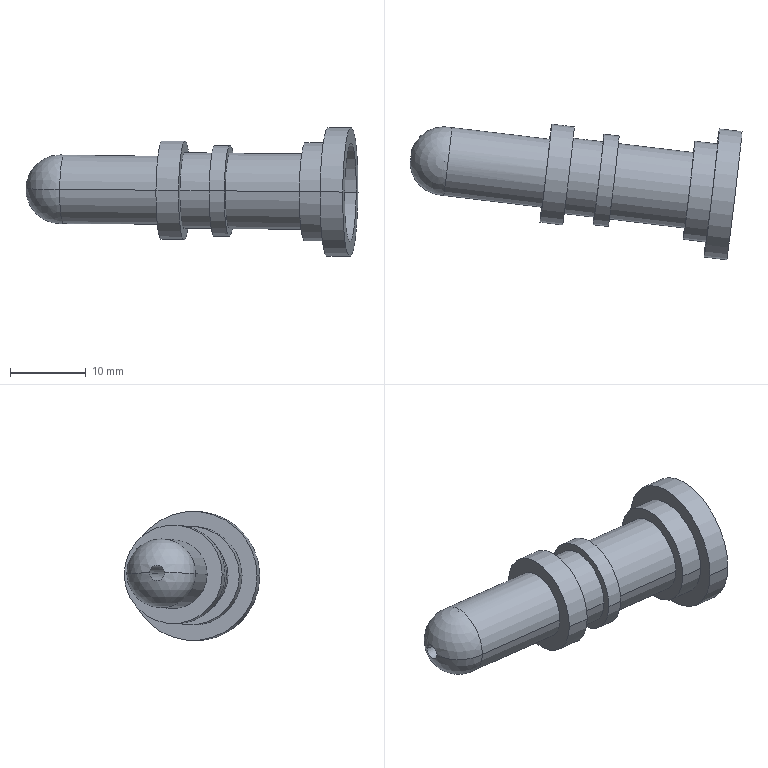Component | SolidWorks | Part12-1 | 1 solid | 29 faces | box 43.71 x 17.85 x 17.03 mm | volume 3533 mm3 | cylinder 18 | plane 9 | sphere 2 | commonest cylinder face diameters 13 x6 10 x4 2 x2 9 x2 12 x2 17 x2 | material 45
build123d program:
from build123d import *

# Parameters (mm, degrees)
SKETCH1_R                = 5
BOSS_EXTRUDE1_DEPTH      = 3
SKETCH2_R                = 6.5
BOSS_EXTRUDE2_DEPTH      = 4
BOSS_EXTRUDE3_DEPTH      = 2
BOSS_EXTRUDE3_DEPTH_BACK = 1
SKETCH3_R                = 8.5
SKETCH3_R_2              = 6.5
SKETCH4_R                = 5
BOSS_EXTRUDE4_DEPTH      = 9
SKETCH5_R                = 6
BOSS_EXTRUDE5_DEPTH      = 2
SKETCH7_R                = 5
BOSS_EXTRUDE6_DEPTH      = 4
BOSS_EXTRUDE7_START      = 3
SKETCH8_R                = 6.5
BOSS_EXTRUDE7_DEPTH      = 3
SKETCH10_R               = 4.5
BOSS_EXTRUDE8_DEPTH      = 13
DOME1_FACE_RADIUS        = 4.5
DOME1_HEIGHT             = 5
SKETCH11_R               = 1
CUT_EXTRUDE1_DEPTH       = 26


with BuildPart() as part:
    # Sketch1 → Boss-Extrude1 (new body)
    with BuildSketch(Plane.XY):
        with Locations((3, 0)):
            Circle(SKETCH1_R)
    extrude(amount=-BOSS_EXTRUDE1_DEPTH)

    # Sketch2 → Boss-Extrude2 (add)
    with BuildSketch(Plane.XY):
        with Locations((3, 0)):
            Circle(SKETCH2_R)
    extrude(amount=BOSS_EXTRUDE2_DEPTH)

    # Sketch3 → Boss-Extrude3 (add, two sides: drawn at the far end of the back side and taken through both)
    with BuildSketch(Plane.XY.offset(4).offset(-BOSS_EXTRUDE3_DEPTH_BACK)):
        with Locations((3, 0)):
            Circle(SKETCH3_R)
        with Locations((3, 0)):
            Circle(SKETCH3_R_2, mode=Mode.SUBTRACT)
    extrude(amount=BOSS_EXTRUDE3_DEPTH + BOSS_EXTRUDE3_DEPTH_BACK)

    # Sketch4 → Boss-Extrude4 (add)
    with BuildSketch(Plane(origin=(0, 0, -3), x_dir=(-1, 0, 0), z_dir=(0, 0, -1))):
        with Locations(Location((-3, 0, 0), (0, 0, 180))):
            Circle(SKETCH4_R)
    extrude(amount=BOSS_EXTRUDE4_DEPTH)

    # Sketch5 → Boss-Extrude5 (add)
    with BuildSketch(Plane(origin=(0, 0, -12), x_dir=(-1, 0, 0), z_dir=(0, 0, -1))):
        with Locations((-3, 0)):
            Circle(SKETCH5_R)
    extrude(amount=-BOSS_EXTRUDE5_DEPTH)

    # Sketch7 → Boss-Extrude6 (add)
    with BuildSketch(Plane(origin=(0, 0, -12), x_dir=(-1, 0, 0), z_dir=(0, 0, -1))):
        with Locations(Location((-3, 0, 0), (0, 0, 180))):
            Circle(SKETCH7_R)
    extrude(amount=BOSS_EXTRUDE6_DEPTH)

    # Sketch8 → Boss-Extrude7 (add)
    with BuildSketch(Plane(origin=(0, 0, -16), x_dir=(-1, 0, 0), z_dir=(0, 0, -1)).offset(BOSS_EXTRUDE7_START)):
        with Locations(Location((-3, 0, 0), (0, 0, 180))):
            Circle(SKETCH8_R)
    extrude(amount=-BOSS_EXTRUDE7_DEPTH)

    # Sketch10 → Boss-Extrude8 (add)
    with BuildSketch(Plane(origin=(0, 0, -19), x_dir=(-1, 0, 0), z_dir=(0, 0, -1))):
        with Locations((-3, 0)):
            Circle(SKETCH10_R)
    extrude(amount=BOSS_EXTRUDE8_DEPTH)

    # Dome1: a dome of height H over a round flat face of radius A is a cap of a sphere of radius (A * A + H * H) / (2 * H)
    dome1_r = (DOME1_FACE_RADIUS * DOME1_FACE_RADIUS + DOME1_HEIGHT * DOME1_HEIGHT) / (2 * DOME1_HEIGHT)
    dome1_base = Plane((3, 0, -32), z_dir=(0, 0, -1))
    with Locations(dome1_base.offset(DOME1_HEIGHT - dome1_r)):
        dome1_ball = Sphere(dome1_r, mode=Mode.PRIVATE)
    add(split(dome1_ball, bisect_by=dome1_base, keep=Keep.TOP, mode=Mode.PRIVATE))

    # Sketch11 → Cut-Extrude1 (cut)
    with BuildSketch(Plane(origin=(0, 0, -19), x_dir=(-1, 0, 0), z_dir=(0, 0, -1))):
        with Locations(Location((-3, 0, 0), (0, 0, 180))):
            Circle(SKETCH11_R)
    extrude(amount=CUT_EXTRUDE1_DEPTH, mode=Mode.SUBTRACT)


solid = part.part

# Placed as in the assembly
solid = solid.moved(Location((7.17, 63.338, -1.925), (94.698, 83.182, -4.568)))
STEP:
#1=COLOUR_RGB('',0.7922,0.8196,0.9333);
#2=FILL_AREA_STYLE_COLOUR('',#1);
#3=FILL_AREA_STYLE('',(#2));
#4=SURFACE_STYLE_FILL_AREA(#3);
#5=SURFACE_SIDE_STYLE('',(#4));
#6=SURFACE_STYLE_USAGE(.BOTH.,#5);
#7=PRESENTATION_STYLE_ASSIGNMENT((#6));
#8=CARTESIAN_POINT('',(-1.141,2.822,-0.0615));
#9=VERTEX_POINT('',#8);
#10=CARTESIAN_POINT('',(-1.15,2.744,-0.06141));
#11=VERTEX_POINT('',#10);
#12=CARTESIAN_POINT('',(-1.146,2.783,-0.06145));
#13=DIRECTION('',(0.9929,-0.1183,-0.009724));
#14=DIRECTION('',(-0.1183,-0.993,0.001159));
#15=AXIS2_PLACEMENT_3D('',#12,#13,#14);
#16=CIRCLE('',#15,0.03937);
#17=EDGE_CURVE('',#9,#11,#16,.T.);
#18=ORIENTED_EDGE('',*,*,#17,.F.);
#19=CARTESIAN_POINT('',(-0.4418,2.738,-0.06835));
#20=VERTEX_POINT('',#19);
#21=CARTESIAN_POINT('',(-1.458,2.86,-0.05839));
#22=DIRECTION('',(0.9929,-0.1183,-0.009724));
#23=VECTOR('',#22,39.37);
#24=LINE('',#21,#23);
#25=EDGE_CURVE('',#9,#20,#24,.T.);
#26=ORIENTED_EDGE('',*,*,#25,.T.);
#27=CARTESIAN_POINT('',(-0.4511,2.66,-0.06826));
#28=VERTEX_POINT('',#27);
#29=CARTESIAN_POINT('',(-0.4465,2.699,-0.0683));
#30=DIRECTION('',(-0.9929,0.1183,0.009724));
#31=DIRECTION('',(0.1183,0.993,-0.001159));
#32=AXIS2_PLACEMENT_3D('',#29,#30,#31);
#33=CIRCLE('',#32,0.03937);
#34=EDGE_CURVE('',#28,#20,#33,.T.);
#35=ORIENTED_EDGE('',*,*,#34,.F.);
#36=CARTESIAN_POINT('',(-1.468,2.781,-0.0583));
#37=DIRECTION('',(0.9929,-0.1183,-0.009724));
#38=VECTOR('',#37,39.37);
#39=LINE('',#36,#38);
#40=EDGE_CURVE('',#11,#28,#39,.T.);
#41=ORIENTED_EDGE('',*,*,#40,.F.);
#42=EDGE_LOOP('',(#18,#26,#35,#41));
#43=FACE_OUTER_BOUND('',#42,.T.);
#44=CARTESIAN_POINT('',(-1.463,2.821,-0.05835));
#45=DIRECTION('',(0.9929,-0.1183,-0.009724));
#46=DIRECTION('',(-0.1183,-0.993,0.001159));
#47=AXIS2_PLACEMENT_3D('',#44,#45,#46);
#48=CYLINDRICAL_SURFACE('',#47,0.03937);
#49=ADVANCED_FACE('',(#43),#48,.F.);
#50=CARTESIAN_POINT('',(-0.9337,2.936,-0.06353));
#51=VERTEX_POINT('',#50);
#52=CARTESIAN_POINT('',(-0.9756,2.584,-0.06312));
#53=VERTEX_POINT('',#52);
#54=CARTESIAN_POINT('',(-0.9547,2.76,-0.06333));
#55=DIRECTION('',(-0.9929,0.1183,0.009724));
#56=DIRECTION('',(0.1183,0.993,-0.001159));
#57=AXIS2_PLACEMENT_3D('',#54,#55,#56);
#58=CIRCLE('',#57,0.1772);
#59=EDGE_CURVE('',#51,#53,#58,.T.);
#60=ORIENTED_EDGE('',*,*,#59,.F.);
#61=CARTESIAN_POINT('',(-0.4255,2.875,-0.06851));
#62=VERTEX_POINT('',#61);
#63=CARTESIAN_POINT('',(-0.9337,2.936,-0.06353));
#64=DIRECTION('',(0.9929,-0.1183,-0.009724));
#65=VECTOR('',#64,39.37);
#66=LINE('',#63,#65);
#67=EDGE_CURVE('',#51,#62,#66,.T.);
#68=ORIENTED_EDGE('',*,*,#67,.T.);
#69=CARTESIAN_POINT('',(-0.4674,2.523,-0.0681));
#70=VERTEX_POINT('',#69);
#71=CARTESIAN_POINT('',(-0.4465,2.699,-0.0683));
#72=DIRECTION('',(-0.9929,0.1183,0.009724));
#73=DIRECTION('',(0.1183,0.993,-0.001159));
#74=AXIS2_PLACEMENT_3D('',#71,#72,#73);
#75=CIRCLE('',#74,0.1772);
#76=EDGE_CURVE('',#62,#70,#75,.T.);
#77=ORIENTED_EDGE('',*,*,#76,.T.);
#78=CARTESIAN_POINT('',(-0.9756,2.584,-0.06312));
#79=DIRECTION('',(0.9929,-0.1183,-0.009724));
#80=VECTOR('',#79,39.37);
#81=LINE('',#78,#80);
#82=EDGE_CURVE('',#53,#70,#81,.T.);
#83=ORIENTED_EDGE('',*,*,#82,.F.);
#84=EDGE_LOOP('',(#60,#68,#77,#83));
#85=FACE_OUTER_BOUND('',#84,.T.);
#86=CARTESIAN_POINT('',(-0.9547,2.76,-0.06333));
#87=DIRECTION('',(0.9929,-0.1183,-0.009724));
#88=DIRECTION('',(-0.1183,-0.993,0.001159));
#89=AXIS2_PLACEMENT_3D('',#86,#87,#88);
#90=CYLINDRICAL_SURFACE('',#89,0.1772);
#91=ADVANCED_FACE('',(#85),#90,.T.);
#92=CARTESIAN_POINT('',(-0.4162,2.954,-0.0686));
#93=VERTEX_POINT('',#92);
#94=CARTESIAN_POINT('',(-0.4767,2.445,-0.06801));
#95=VERTEX_POINT('',#94);
#96=CARTESIAN_POINT('',(-0.4465,2.699,-0.0683));
#97=DIRECTION('',(-0.9929,0.1183,0.009724));
#98=DIRECTION('',(0.1183,0.993,-0.001159));
#99=AXIS2_PLACEMENT_3D('',#96,#97,#98);
#100=CIRCLE('',#99,0.2559);
#101=EDGE_CURVE('',#93,#95,#100,.T.);
#102=ORIENTED_EDGE('',*,*,#101,.F.);
#103=CARTESIAN_POINT('',(-0.2989,2.94,-0.06975));
#104=VERTEX_POINT('',#103);
#105=CARTESIAN_POINT('',(-0.4162,2.954,-0.0686));
#106=DIRECTION('',(0.9929,-0.1183,-0.009724));
#107=VECTOR('',#106,39.37);
#108=LINE('',#105,#107);
#109=EDGE_CURVE('',#93,#104,#108,.T.);
#110=ORIENTED_EDGE('',*,*,#109,.T.);
#111=CARTESIAN_POINT('',(-0.3595,2.431,-0.06915));
#112=VERTEX_POINT('',#111);
#113=CARTESIAN_POINT('',(-0.3292,2.685,-0.06945));
#114=DIRECTION('',(-0.9929,0.1183,0.009724));
#115=DIRECTION('',(0.1183,0.993,-0.001159));
#116=AXIS2_PLACEMENT_3D('',#113,#114,#115);
#117=CIRCLE('',#116,0.2559);
#118=EDGE_CURVE('',#104,#112,#117,.T.);
#119=ORIENTED_EDGE('',*,*,#118,.T.);
#120=CARTESIAN_POINT('',(-0.4767,2.445,-0.06801));
#121=DIRECTION('',(0.9929,-0.1183,-0.009724));
#122=VECTOR('',#121,39.37);
#123=LINE('',#120,#122);
#124=EDGE_CURVE('',#95,#112,#123,.T.);
#125=ORIENTED_EDGE('',*,*,#124,.F.);
#126=EDGE_LOOP('',(#102,#110,#119,#125));
#127=FACE_OUTER_BOUND('',#126,.T.);
#128=CARTESIAN_POINT('',(-0.4465,2.699,-0.0683));
#129=DIRECTION('',(0.9929,-0.1183,-0.009724));
#130=DIRECTION('',(-0.1183,-0.993,0.001159));
#131=AXIS2_PLACEMENT_3D('',#128,#129,#130);
#132=CYLINDRICAL_SURFACE('',#131,0.2559);
#133=ADVANCED_FACE('',(#127),#132,.T.);
#134=CARTESIAN_POINT('',(-0.3059,2.881,-0.06968));
#135=VERTEX_POINT('',#134);
#136=CARTESIAN_POINT('',(-0.3525,2.49,-0.06922));
#137=VERTEX_POINT('',#136);
#138=CARTESIAN_POINT('',(-0.3292,2.685,-0.06945));
#139=DIRECTION('',(-0.9929,0.1183,0.009724));
#140=DIRECTION('',(0.1183,0.993,-0.001159));
#141=AXIS2_PLACEMENT_3D('',#138,#139,#140);
#142=CIRCLE('',#141,0.1969);
#143=EDGE_CURVE('',#135,#137,#142,.T.);
#144=ORIENTED_EDGE('',*,*,#143,.F.);
#145=CARTESIAN_POINT('',(-0.1495,2.862,-0.07121));
#146=VERTEX_POINT('',#145);
#147=CARTESIAN_POINT('',(-0.3059,2.881,-0.06968));
#148=DIRECTION('',(0.9929,-0.1183,-0.009724));
#149=VECTOR('',#148,39.37);
#150=LINE('',#147,#149);
#151=EDGE_CURVE('',#135,#146,#150,.T.);
#152=ORIENTED_EDGE('',*,*,#151,.T.);
#153=CARTESIAN_POINT('',(-0.1961,2.471,-0.07075));
#154=VERTEX_POINT('',#153);
#155=CARTESIAN_POINT('',(-0.1728,2.667,-0.07098));
#156=DIRECTION('',(-0.9929,0.1183,0.009724));
#157=DIRECTION('',(0.1183,0.993,-0.001159));
#158=AXIS2_PLACEMENT_3D('',#155,#156,#157);
#159=CIRCLE('',#158,0.1969);
#160=EDGE_CURVE('',#146,#154,#159,.T.);
#161=ORIENTED_EDGE('',*,*,#160,.T.);
#162=CARTESIAN_POINT('',(-0.3525,2.49,-0.06922));
#163=DIRECTION('',(0.9929,-0.1183,-0.009724));
#164=VECTOR('',#163,39.37);
#165=LINE('',#162,#164);
#166=EDGE_CURVE('',#137,#154,#165,.T.);
#167=ORIENTED_EDGE('',*,*,#166,.F.);
#168=EDGE_LOOP('',(#144,#152,#161,#167));
#169=FACE_OUTER_BOUND('',#168,.T.);
#170=CARTESIAN_POINT('',(-0.3292,2.685,-0.06945));
#171=DIRECTION('',(0.9929,-0.1183,-0.009724));
#172=DIRECTION('',(-0.1183,-0.993,0.001159));
#173=AXIS2_PLACEMENT_3D('',#170,#171,#172);
#174=CYLINDRICAL_SURFACE('',#173,0.1969);
#175=ADVANCED_FACE('',(#169),#174,.T.);
#176=CARTESIAN_POINT('',(-0.06669,2.892,-0.07202));
#177=VERTEX_POINT('',#176);
#178=CARTESIAN_POINT('',(-0.1226,2.423,-0.07147));
#179=VERTEX_POINT('',#178);
#180=CARTESIAN_POINT('',(-0.09464,2.657,-0.07175));
#181=DIRECTION('',(-0.9929,0.1183,0.009724));
#182=DIRECTION('',(0.1183,0.993,-0.001159));
#183=AXIS2_PLACEMENT_3D('',#180,#181,#182);
#184=CIRCLE('',#183,0.2362);
#185=EDGE_CURVE('',#177,#179,#184,.T.);
#186=ORIENTED_EDGE('',*,*,#185,.T.);
#187=CARTESIAN_POINT('',(-0.2008,2.432,-0.07071));
#188=VERTEX_POINT('',#187);
#189=CARTESIAN_POINT('',(-0.1226,2.423,-0.07147));
#190=DIRECTION('',(-0.9929,0.1183,0.009724));
#191=VECTOR('',#190,39.37);
#192=LINE('',#189,#191);
#193=EDGE_CURVE('',#179,#188,#192,.T.);
#194=ORIENTED_EDGE('',*,*,#193,.T.);
#195=CARTESIAN_POINT('',(-0.1449,2.901,-0.07126));
#196=VERTEX_POINT('',#195);
#197=CARTESIAN_POINT('',(-0.1728,2.667,-0.07098));
#198=DIRECTION('',(-0.9929,0.1183,0.009724));
#199=DIRECTION('',(0.1183,0.993,-0.001159));
#200=AXIS2_PLACEMENT_3D('',#197,#198,#199);
#201=CIRCLE('',#200,0.2362);
#202=EDGE_CURVE('',#196,#188,#201,.T.);
#203=ORIENTED_EDGE('',*,*,#202,.F.);
#204=CARTESIAN_POINT('',(-0.06669,2.892,-0.07202));
#205=DIRECTION('',(-0.9929,0.1183,0.009724));
#206=VECTOR('',#205,39.37);
#207=LINE('',#204,#206);
#208=EDGE_CURVE('',#177,#196,#207,.T.);
#209=ORIENTED_EDGE('',*,*,#208,.F.);
#210=EDGE_LOOP('',(#186,#194,#203,#209));
#211=FACE_OUTER_BOUND('',#210,.T.);
#212=CARTESIAN_POINT('',(-0.09464,2.657,-0.07175));
#213=DIRECTION('',(-0.9929,0.1183,0.009724));
#214=DIRECTION('',(0.1183,0.993,-0.001159));
#215=AXIS2_PLACEMENT_3D('',#212,#213,#214);
#216=CYLINDRICAL_SURFACE('',#215,0.2362);
#217=ADVANCED_FACE('',(#211),#216,.T.);
#218=CARTESIAN_POINT('',(0.4829,2.846,-0.07741));
#219=VERTEX_POINT('',#218);
#220=CARTESIAN_POINT('',(0.4224,2.338,-0.07681));
#221=VERTEX_POINT('',#220);
#222=CARTESIAN_POINT('',(0.4526,2.592,-0.07711));
#223=DIRECTION('',(0.9929,-0.1183,-0.009724));
#224=DIRECTION('',(-0.1183,-0.993,0.001159));
#225=AXIS2_PLACEMENT_3D('',#222,#223,#224);
#226=CIRCLE('',#225,0.2559);
#227=EDGE_CURVE('',#219,#221,#226,.T.);
#228=ORIENTED_EDGE('',*,*,#227,.F.);
#229=CARTESIAN_POINT('',(0.5611,2.837,-0.07817));
#230=VERTEX_POINT('',#229);
#231=CARTESIAN_POINT('',(0.4438,2.851,-0.07702));
#232=DIRECTION('',(0.9929,-0.1183,-0.009724));
#233=VECTOR('',#232,39.37);
#234=LINE('',#231,#233);
#235=EDGE_CURVE('',#219,#230,#234,.T.);
#236=ORIENTED_EDGE('',*,*,#235,.T.);
#237=CARTESIAN_POINT('',(0.5005,2.329,-0.07758));
#238=VERTEX_POINT('',#237);
#239=CARTESIAN_POINT('',(0.5308,2.583,-0.07787));
#240=DIRECTION('',(0.9929,-0.1183,-0.009724));
#241=DIRECTION('',(-0.1183,-0.993,0.001159));
#242=AXIS2_PLACEMENT_3D('',#239,#240,#241);
#243=CIRCLE('',#242,0.2559);
#244=EDGE_CURVE('',#230,#238,#243,.T.);
#245=ORIENTED_EDGE('',*,*,#244,.T.);
#246=CARTESIAN_POINT('',(0.3833,2.343,-0.07643));
#247=DIRECTION('',(0.9929,-0.1183,-0.009724));
#248=VECTOR('',#247,39.37);
#249=LINE('',#246,#248);
#250=EDGE_CURVE('',#221,#238,#249,.T.);
#251=ORIENTED_EDGE('',*,*,#250,.F.);
#252=EDGE_LOOP('',(#228,#236,#245,#251));
#253=FACE_OUTER_BOUND('',#252,.T.);
#254=CARTESIAN_POINT('',(0.4136,2.597,-0.07673));
#255=DIRECTION('',(0.9929,-0.1183,-0.009724));
#256=DIRECTION('',(-0.1183,-0.993,0.001159));
#257=AXIS2_PLACEMENT_3D('',#254,#255,#256);
#258=CYLINDRICAL_SURFACE('',#257,0.2559);
#259=ADVANCED_FACE('',(#253),#258,.F.);
#260=CARTESIAN_POINT('',(0.374,2.265,-0.07634));
#261=VERTEX_POINT('',#260);
#262=CARTESIAN_POINT('',(0.4531,2.929,-0.07711));
#263=VERTEX_POINT('',#262);
#264=CARTESIAN_POINT('',(0.4136,2.597,-0.07673));
#265=DIRECTION('',(0.9929,-0.1183,-0.009724));
#266=DIRECTION('',(-0.1183,-0.993,0.001159));
#267=AXIS2_PLACEMENT_3D('',#264,#265,#266);
#268=CIRCLE('',#267,0.3346);
#269=EDGE_CURVE('',#261,#263,#268,.T.);
#270=ORIENTED_EDGE('',*,*,#269,.T.);
#271=CARTESIAN_POINT('',(0.5704,2.915,-0.07826));
#272=VERTEX_POINT('',#271);
#273=CARTESIAN_POINT('',(0.4531,2.929,-0.07711));
#274=DIRECTION('',(0.9929,-0.1183,-0.009724));
#275=VECTOR('',#274,39.37);
#276=LINE('',#273,#275);
#277=EDGE_CURVE('',#263,#272,#276,.T.);
#278=ORIENTED_EDGE('',*,*,#277,.T.);
#279=CARTESIAN_POINT('',(0.4912,2.251,-0.07749));
#280=VERTEX_POINT('',#279);
#281=CARTESIAN_POINT('',(0.5308,2.583,-0.07787));
#282=DIRECTION('',(0.9929,-0.1183,-0.009724));
#283=DIRECTION('',(-0.1183,-0.993,0.001159));
#284=AXIS2_PLACEMENT_3D('',#281,#282,#283);
#285=CIRCLE('',#284,0.3346);
#286=EDGE_CURVE('',#280,#272,#285,.T.);
#287=ORIENTED_EDGE('',*,*,#286,.F.);
#288=CARTESIAN_POINT('',(0.374,2.265,-0.07634));
#289=DIRECTION('',(0.9929,-0.1183,-0.009724));
#290=VECTOR('',#289,39.37);
#291=LINE('',#288,#290);
#292=EDGE_CURVE('',#261,#280,#291,.T.);
#293=ORIENTED_EDGE('',*,*,#292,.F.);
#294=EDGE_LOOP('',(#270,#278,#287,#293));
#295=FACE_OUTER_BOUND('',#294,.T.);
#296=CARTESIAN_POINT('',(0.4136,2.597,-0.07673));
#297=DIRECTION('',(0.9929,-0.1183,-0.009724));
#298=DIRECTION('',(-0.1183,-0.993,0.001159));
#299=AXIS2_PLACEMENT_3D('',#296,#297,#298);
#300=CYLINDRICAL_SURFACE('',#299,0.3346);
#301=ADVANCED_FACE('',(#295),#300,.T.);
#302=CARTESIAN_POINT('',(0.3833,2.343,-0.07643));
#303=VERTEX_POINT('',#302);
#304=CARTESIAN_POINT('',(0.4438,2.851,-0.07702));
#305=VERTEX_POINT('',#304);
#306=CARTESIAN_POINT('',(0.4136,2.597,-0.07673));
#307=DIRECTION('',(0.9929,-0.1183,-0.009724));
#308=DIRECTION('',(-0.1183,-0.993,0.001159));
#309=AXIS2_PLACEMENT_3D('',#306,#307,#308);
#310=CIRCLE('',#309,0.2559);
#311=EDGE_CURVE('',#303,#305,#310,.T.);
#312=ORIENTED_EDGE('',*,*,#311,.F.);
#313=CARTESIAN_POINT('',(0.266,2.357,-0.07528));
#314=VERTEX_POINT('',#313);
#315=CARTESIAN_POINT('',(0.4224,2.338,-0.07681));
#316=DIRECTION('',(-0.9929,0.1183,0.009724));
#317=VECTOR('',#316,39.37);
#318=LINE('',#315,#317);
#319=EDGE_CURVE('',#303,#314,#318,.T.);
#320=ORIENTED_EDGE('',*,*,#319,.T.);
#321=CARTESIAN_POINT('',(0.3266,2.865,-0.07587));
#322=VERTEX_POINT('',#321);
#323=CARTESIAN_POINT('',(0.2963,2.611,-0.07558));
#324=DIRECTION('',(0.9929,-0.1183,-0.009724));
#325=DIRECTION('',(-0.1183,-0.993,0.001159));
#326=AXIS2_PLACEMENT_3D('',#323,#324,#325);
#327=CIRCLE('',#326,0.2559);
#328=EDGE_CURVE('',#314,#322,#327,.T.);
#329=ORIENTED_EDGE('',*,*,#328,.T.);
#330=CARTESIAN_POINT('',(0.4829,2.846,-0.07741));
#331=DIRECTION('',(-0.9929,0.1183,0.009724));
#332=VECTOR('',#331,39.37);
#333=LINE('',#330,#332);
#334=EDGE_CURVE('',#305,#322,#333,.T.);
#335=ORIENTED_EDGE('',*,*,#334,.F.);
#336=EDGE_LOOP('',(#312,#320,#329,#335));
#337=FACE_OUTER_BOUND('',#336,.T.);
#338=CARTESIAN_POINT('',(0.4526,2.592,-0.07711));
#339=DIRECTION('',(-0.9929,0.1183,0.009724));
#340=DIRECTION('',(0.1183,0.993,-0.001159));
#341=AXIS2_PLACEMENT_3D('',#338,#339,#340);
#342=CYLINDRICAL_SURFACE('',#341,0.2559);
#343=ADVANCED_FACE('',(#337),#342,.T.);
#344=CARTESIAN_POINT('',(-0.1179,2.462,-0.07152));
#345=VERTEX_POINT('',#344);
#346=CARTESIAN_POINT('',(-0.07135,2.853,-0.07198));
#347=VERTEX_POINT('',#346);
#348=CARTESIAN_POINT('',(-0.09464,2.657,-0.07175));
#349=DIRECTION('',(0.9929,-0.1183,-0.009724));
#350=DIRECTION('',(0.1183,0.993,-0.001159));
#351=AXIS2_PLACEMENT_3D('',#348,#349,#350);
#352=CIRCLE('',#351,0.1969);
#353=EDGE_CURVE('',#345,#347,#352,.T.);
#354=ORIENTED_EDGE('',*,*,#353,.T.);
#355=CARTESIAN_POINT('',(0.3196,2.806,-0.07581));
#356=VERTEX_POINT('',#355);
#357=CARTESIAN_POINT('',(0.2023,2.82,-0.07466));
#358=DIRECTION('',(0.9929,-0.1183,-0.009724));
#359=VECTOR('',#358,39.37);
#360=LINE('',#357,#359);
#361=EDGE_CURVE('',#347,#356,#360,.T.);
#362=ORIENTED_EDGE('',*,*,#361,.T.);
#363=CARTESIAN_POINT('',(0.273,2.415,-0.07535));
#364=VERTEX_POINT('',#363);
#365=CARTESIAN_POINT('',(0.2963,2.611,-0.07558));
#366=DIRECTION('',(0.9929,-0.1183,-0.009724));
#367=DIRECTION('',(-0.1183,-0.993,0.001159));
#368=AXIS2_PLACEMENT_3D('',#365,#366,#367);
#369=CIRCLE('',#368,0.1969);
#370=EDGE_CURVE('',#364,#356,#369,.T.);
#371=ORIENTED_EDGE('',*,*,#370,.F.);
#372=CARTESIAN_POINT('',(0.1557,2.429,-0.0742));
#373=DIRECTION('',(0.9929,-0.1183,-0.009724));
#374=VECTOR('',#373,39.37);
#375=LINE('',#372,#374);
#376=EDGE_CURVE('',#345,#364,#375,.T.);
#377=ORIENTED_EDGE('',*,*,#376,.F.);
#378=EDGE_LOOP('',(#354,#362,#371,#377));
#379=FACE_OUTER_BOUND('',#378,.T.);
#380=CARTESIAN_POINT('',(0.179,2.625,-0.07443));
#381=DIRECTION('',(0.9929,-0.1183,-0.009724));
#382=DIRECTION('',(-0.1183,-0.993,0.001159));
#383=AXIS2_PLACEMENT_3D('',#380,#381,#382);
#384=CYLINDRICAL_SURFACE('',#383,0.1969);
#385=ADVANCED_FACE('',(#379),#384,.T.);
#386=CARTESIAN_POINT('',(-1.146,2.783,-0.06145));
#387=DIRECTION('',(0.9929,-0.1183,-0.009724));
#388=DIRECTION('',(-0.1183,-0.993,0.001159));
#389=AXIS2_PLACEMENT_3D('',#386,#387,#388);
#390=CIRCLE('',#389,0.03937);
#391=EDGE_CURVE('',#11,#9,#390,.T.);
#392=ORIENTED_EDGE('',*,*,#391,.T.);
#393=CARTESIAN_POINT('',(-0.9732,2.762,-0.06314));
#394=DIRECTION('',(-0.009793,-0.,-1.));
#395=DIRECTION('',(-1.,0.,0.009793));
#396=AXIS2_PLACEMENT_3D('',#393,#394,#395);
#397=CIRCLE('',#396,0.1781);
#398=EDGE_CURVE('',#9,#51,#397,.T.);
#399=ORIENTED_EDGE('',*,*,#398,.T.);
#400=ORIENTED_EDGE('',*,*,#59,.T.);
#401=CARTESIAN_POINT('',(-0.9732,2.762,-0.06314));
#402=DIRECTION('',(0.009793,0.,1.));
#403=DIRECTION('',(1.,0.,-0.009793));
#404=AXIS2_PLACEMENT_3D('',#401,#402,#403);
#405=CIRCLE('',#404,0.1781);
#406=EDGE_CURVE('',#11,#53,#405,.T.);
#407=ORIENTED_EDGE('',*,*,#406,.F.);
#408=EDGE_LOOP('',(#392,#399,#400,#407));
#409=FACE_OUTER_BOUND('',#408,.T.);
#410=CARTESIAN_POINT('',(-0.9732,2.762,-0.06314));
#411=DIRECTION('',(-0.009793,-0.,-1.));
#412=DIRECTION('',(-0.1183,-0.993,0.001159));
#413=AXIS2_PLACEMENT_3D('',#410,#411,#412);
#414=SPHERICAL_SURFACE('',#413,0.1781);
#415=ADVANCED_FACE('',(#409),#414,.T.);
#416=ORIENTED_EDGE('',*,*,#398,.F.);
#417=ORIENTED_EDGE('',*,*,#17,.T.);
#418=ORIENTED_EDGE('',*,*,#406,.T.);
#419=CARTESIAN_POINT('',(-0.9547,2.76,-0.06333));
#420=DIRECTION('',(-0.9929,0.1183,0.009724));
#421=DIRECTION('',(0.1183,0.993,-0.001159));
#422=AXIS2_PLACEMENT_3D('',#419,#420,#421);
#423=CIRCLE('',#422,0.1772);
#424=EDGE_CURVE('',#53,#51,#423,.T.);
#425=ORIENTED_EDGE('',*,*,#424,.T.);
#426=EDGE_LOOP('',(#416,#417,#418,#425));
#427=FACE_OUTER_BOUND('',#426,.T.);
#428=CARTESIAN_POINT('',(-0.9732,2.762,-0.06314));
#429=DIRECTION('',(-0.009793,-0.,-1.));
#430=DIRECTION('',(-0.1183,-0.993,0.001159));
#431=AXIS2_PLACEMENT_3D('',#428,#429,#430);
#432=SPHERICAL_SURFACE('',#431,0.1781);
#433=ADVANCED_FACE('',(#427),#432,.T.);
#434=CARTESIAN_POINT('',(-0.4465,2.699,-0.0683));
#435=DIRECTION('',(-0.9929,0.1183,0.009724));
#436=DIRECTION('',(0.1183,0.993,-0.001159));
#437=AXIS2_PLACEMENT_3D('',#434,#435,#436);
#438=CIRCLE('',#437,0.2559);
#439=EDGE_CURVE('',#95,#93,#438,.T.);
#440=ORIENTED_EDGE('',*,*,#439,.T.);
#441=ORIENTED_EDGE('',*,*,#101,.T.);
#442=EDGE_LOOP('',(#440,#441));
#443=FACE_OUTER_BOUND('',#442,.T.);
#444=CARTESIAN_POINT('',(-0.4465,2.699,-0.0683));
#445=DIRECTION('',(-0.9929,0.1183,0.009724));
#446=DIRECTION('',(0.1183,0.993,-0.001159));
#447=AXIS2_PLACEMENT_3D('',#444,#445,#446);
#448=CIRCLE('',#447,0.1772);
#449=EDGE_CURVE('',#70,#62,#448,.T.);
#450=ORIENTED_EDGE('',*,*,#449,.F.);
#451=ORIENTED_EDGE('',*,*,#76,.F.);
#452=EDGE_LOOP('',(#450,#451));
#453=FACE_BOUND('',#452,.T.);
#454=CARTESIAN_POINT('',(-0.4465,2.699,-0.0683));
#455=DIRECTION('',(-0.9929,0.1183,0.009724));
#456=DIRECTION('',(0.1183,0.993,-0.001159));
#457=AXIS2_PLACEMENT_3D('',#454,#455,#456);
#458=PLANE('',#457);
#459=ADVANCED_FACE('',(#443,#453),#458,.T.);
#460=ORIENTED_EDGE('',*,*,#202,.T.);
#461=CARTESIAN_POINT('',(-0.1728,2.667,-0.07098));
#462=DIRECTION('',(-0.9929,0.1183,0.009724));
#463=DIRECTION('',(0.1183,0.993,-0.001159));
#464=AXIS2_PLACEMENT_3D('',#461,#462,#463);
#465=CIRCLE('',#464,0.2362);
#466=EDGE_CURVE('',#188,#196,#465,.T.);
#467=ORIENTED_EDGE('',*,*,#466,.T.);
#468=EDGE_LOOP('',(#460,#467));
#469=FACE_OUTER_BOUND('',#468,.T.);
#470=CARTESIAN_POINT('',(-0.1728,2.667,-0.07098));
#471=DIRECTION('',(-0.9929,0.1183,0.009724));
#472=DIRECTION('',(0.1183,0.993,-0.001159));
#473=AXIS2_PLACEMENT_3D('',#470,#471,#472);
#474=CIRCLE('',#473,0.1969);
#475=EDGE_CURVE('',#154,#146,#474,.T.);
#476=ORIENTED_EDGE('',*,*,#475,.F.);
#477=ORIENTED_EDGE('',*,*,#160,.F.);
#478=EDGE_LOOP('',(#476,#477));
#479=FACE_BOUND('',#478,.T.);
#480=CARTESIAN_POINT('',(-0.1728,2.667,-0.07098));
#481=DIRECTION('',(-0.9929,0.1183,0.009724));
#482=DIRECTION('',(0.1183,0.993,-0.001159));
#483=AXIS2_PLACEMENT_3D('',#480,#481,#482);
#484=PLANE('',#483);
#485=ADVANCED_FACE('',(#469,#479),#484,.T.);
#486=ORIENTED_EDGE('',*,*,#361,.F.);
#487=CARTESIAN_POINT('',(-0.09464,2.657,-0.07175));
#488=DIRECTION('',(0.9929,-0.1183,-0.009724));
#489=DIRECTION('',(0.1183,0.993,-0.001159));
#490=AXIS2_PLACEMENT_3D('',#487,#488,#489);
#491=CIRCLE('',#490,0.1969);
#492=EDGE_CURVE('',#347,#345,#491,.T.);
#493=ORIENTED_EDGE('',*,*,#492,.T.);
#494=ORIENTED_EDGE('',*,*,#376,.T.);
#495=CARTESIAN_POINT('',(0.2963,2.611,-0.07558));
#496=DIRECTION('',(0.9929,-0.1183,-0.009724));
#497=DIRECTION('',(-0.1183,-0.993,0.001159));
#498=AXIS2_PLACEMENT_3D('',#495,#496,#497);
#499=CIRCLE('',#498,0.1969);
#500=EDGE_CURVE('',#356,#364,#499,.T.);
#501=ORIENTED_EDGE('',*,*,#500,.F.);
#502=EDGE_LOOP('',(#486,#493,#494,#501));
#503=FACE_OUTER_BOUND('',#502,.T.);
#504=CARTESIAN_POINT('',(0.179,2.625,-0.07443));
#505=DIRECTION('',(0.9929,-0.1183,-0.009724));
#506=DIRECTION('',(-0.1183,-0.993,0.001159));
#507=AXIS2_PLACEMENT_3D('',#504,#505,#506);
#508=CYLINDRICAL_SURFACE('',#507,0.1969);
#509=ADVANCED_FACE('',(#503),#508,.T.);
#510=ORIENTED_EDGE('',*,*,#319,.F.);
#511=CARTESIAN_POINT('',(0.4136,2.597,-0.07673));
#512=DIRECTION('',(0.9929,-0.1183,-0.009724));
#513=DIRECTION('',(-0.1183,-0.993,0.001159));
#514=AXIS2_PLACEMENT_3D('',#511,#512,#513);
#515=CIRCLE('',#514,0.2559);
#516=EDGE_CURVE('',#305,#303,#515,.T.);
#517=ORIENTED_EDGE('',*,*,#516,.F.);
#518=ORIENTED_EDGE('',*,*,#334,.T.);
#519=CARTESIAN_POINT('',(0.2963,2.611,-0.07558));
#520=DIRECTION('',(0.9929,-0.1183,-0.009724));
#521=DIRECTION('',(-0.1183,-0.993,0.001159));
#522=AXIS2_PLACEMENT_3D('',#519,#520,#521);
#523=CIRCLE('',#522,0.2559);
#524=EDGE_CURVE('',#322,#314,#523,.T.);
#525=ORIENTED_EDGE('',*,*,#524,.T.);
#526=EDGE_LOOP('',(#510,#517,#518,#525));
#527=FACE_OUTER_BOUND('',#526,.T.);
#528=CARTESIAN_POINT('',(0.4526,2.592,-0.07711));
#529=DIRECTION('',(-0.9929,0.1183,0.009724));
#530=DIRECTION('',(0.1183,0.993,-0.001159));
#531=AXIS2_PLACEMENT_3D('',#528,#529,#530);
#532=CYLINDRICAL_SURFACE('',#531,0.2559);
#533=ADVANCED_FACE('',(#527),#532,.T.);
#534=ORIENTED_EDGE('',*,*,#370,.T.);
#535=ORIENTED_EDGE('',*,*,#500,.T.);
#536=EDGE_LOOP('',(#534,#535));
#537=FACE_BOUND('',#536,.T.);
#538=ORIENTED_EDGE('',*,*,#524,.F.);
#539=ORIENTED_EDGE('',*,*,#328,.F.);
#540=EDGE_LOOP('',(#538,#539));
#541=FACE_OUTER_BOUND('',#540,.T.);
#542=CARTESIAN_POINT('',(0.2963,2.611,-0.07558));
#543=DIRECTION('',(0.9929,-0.1183,-0.009724));
#544=DIRECTION('',(-0.1183,-0.993,0.001159));
#545=AXIS2_PLACEMENT_3D('',#542,#543,#544);
#546=PLANE('',#545);
#547=ADVANCED_FACE('',(#537,#541),#546,.F.);
#548=ORIENTED_EDGE('',*,*,#277,.F.);
#549=CARTESIAN_POINT('',(0.4136,2.597,-0.07673));
#550=DIRECTION('',(0.9929,-0.1183,-0.009724));
#551=DIRECTION('',(-0.1183,-0.993,0.001159));
#552=AXIS2_PLACEMENT_3D('',#549,#550,#551);
#553=CIRCLE('',#552,0.3346);
#554=EDGE_CURVE('',#263,#261,#553,.T.);
#555=ORIENTED_EDGE('',*,*,#554,.T.);
#556=ORIENTED_EDGE('',*,*,#292,.T.);
#557=CARTESIAN_POINT('',(0.5308,2.583,-0.07787));
#558=DIRECTION('',(0.9929,-0.1183,-0.009724));
#559=DIRECTION('',(-0.1183,-0.993,0.001159));
#560=AXIS2_PLACEMENT_3D('',#557,#558,#559);
#561=CIRCLE('',#560,0.3346);
#562=EDGE_CURVE('',#272,#280,#561,.T.);
#563=ORIENTED_EDGE('',*,*,#562,.F.);
#564=EDGE_LOOP('',(#548,#555,#556,#563));
#565=FACE_OUTER_BOUND('',#564,.T.);
#566=CARTESIAN_POINT('',(0.4136,2.597,-0.07673));
#567=DIRECTION('',(0.9929,-0.1183,-0.009724));
#568=DIRECTION('',(-0.1183,-0.993,0.001159));
#569=AXIS2_PLACEMENT_3D('',#566,#567,#568);
#570=CYLINDRICAL_SURFACE('',#569,0.3346);
#571=ADVANCED_FACE('',(#565),#570,.T.);
#572=ORIENTED_EDGE('',*,*,#516,.T.);
#573=ORIENTED_EDGE('',*,*,#311,.T.);
#574=EDGE_LOOP('',(#572,#573));
#575=FACE_BOUND('',#574,.T.);
#576=ORIENTED_EDGE('',*,*,#269,.F.);
#577=ORIENTED_EDGE('',*,*,#554,.F.);
#578=EDGE_LOOP('',(#576,#577));
#579=FACE_OUTER_BOUND('',#578,.T.);
#580=CARTESIAN_POINT('',(0.4136,2.597,-0.07673));
#581=DIRECTION('',(0.9929,-0.1183,-0.009724));
#582=DIRECTION('',(-0.1183,-0.993,0.001159));
#583=AXIS2_PLACEMENT_3D('',#580,#581,#582);
#584=PLANE('',#583);
#585=ADVANCED_FACE('',(#575,#579),#584,.F.);
#586=ORIENTED_EDGE('',*,*,#235,.F.);
#587=CARTESIAN_POINT('',(0.4526,2.592,-0.07711));
#588=DIRECTION('',(0.9929,-0.1183,-0.009724));
#589=DIRECTION('',(-0.1183,-0.993,0.001159));
#590=AXIS2_PLACEMENT_3D('',#587,#588,#589);
#591=CIRCLE('',#590,0.2559);
#592=EDGE_CURVE('',#221,#219,#591,.T.);
#593=ORIENTED_EDGE('',*,*,#592,.F.);
#594=ORIENTED_EDGE('',*,*,#250,.T.);
#595=CARTESIAN_POINT('',(0.5308,2.583,-0.07787));
#596=DIRECTION('',(0.9929,-0.1183,-0.009724));
#597=DIRECTION('',(-0.1183,-0.993,0.001159));
#598=AXIS2_PLACEMENT_3D('',#595,#596,#597);
#599=CIRCLE('',#598,0.2559);
#600=EDGE_CURVE('',#238,#230,#599,.T.);
#601=ORIENTED_EDGE('',*,*,#600,.T.);
#602=EDGE_LOOP('',(#586,#593,#594,#601));
#603=FACE_OUTER_BOUND('',#602,.T.);
#604=CARTESIAN_POINT('',(0.4136,2.597,-0.07673));
#605=DIRECTION('',(0.9929,-0.1183,-0.009724));
#606=DIRECTION('',(-0.1183,-0.993,0.001159));
#607=AXIS2_PLACEMENT_3D('',#604,#605,#606);
#608=CYLINDRICAL_SURFACE('',#607,0.2559);
#609=ADVANCED_FACE('',(#603),#608,.F.);
#610=ORIENTED_EDGE('',*,*,#286,.T.);
#611=ORIENTED_EDGE('',*,*,#562,.T.);
#612=EDGE_LOOP('',(#610,#611));
#613=FACE_OUTER_BOUND('',#612,.T.);
#614=ORIENTED_EDGE('',*,*,#600,.F.);
#615=ORIENTED_EDGE('',*,*,#244,.F.);
#616=EDGE_LOOP('',(#614,#615));
#617=FACE_BOUND('',#616,.T.);
#618=CARTESIAN_POINT('',(0.5308,2.583,-0.07787));
#619=DIRECTION('',(0.9929,-0.1183,-0.009724));
#620=DIRECTION('',(-0.1183,-0.993,0.001159));
#621=AXIS2_PLACEMENT_3D('',#618,#619,#620);
#622=PLANE('',#621);
#623=ADVANCED_FACE('',(#613,#617),#622,.T.);
#624=ORIENTED_EDGE('',*,*,#592,.T.);
#625=ORIENTED_EDGE('',*,*,#227,.T.);
#626=EDGE_LOOP('',(#624,#625));
#627=FACE_OUTER_BOUND('',#626,.T.);
#628=CARTESIAN_POINT('',(0.4526,2.592,-0.07711));
#629=DIRECTION('',(0.9929,-0.1183,-0.009724));
#630=DIRECTION('',(-0.1183,-0.993,0.001159));
#631=AXIS2_PLACEMENT_3D('',#628,#629,#630);
#632=PLANE('',#631);
#633=ADVANCED_FACE('',(#627),#632,.T.);
#634=ORIENTED_EDGE('',*,*,#193,.F.);
#635=CARTESIAN_POINT('',(-0.09464,2.657,-0.07175));
#636=DIRECTION('',(-0.9929,0.1183,0.009724));
#637=DIRECTION('',(0.1183,0.993,-0.001159));
#638=AXIS2_PLACEMENT_3D('',#635,#636,#637);
#639=CIRCLE('',#638,0.2362);
#640=EDGE_CURVE('',#179,#177,#639,.T.);
#641=ORIENTED_EDGE('',*,*,#640,.T.);
#642=ORIENTED_EDGE('',*,*,#208,.T.);
#643=ORIENTED_EDGE('',*,*,#466,.F.);
#644=EDGE_LOOP('',(#634,#641,#642,#643));
#645=FACE_OUTER_BOUND('',#644,.T.);
#646=CARTESIAN_POINT('',(-0.09464,2.657,-0.07175));
#647=DIRECTION('',(-0.9929,0.1183,0.009724));
#648=DIRECTION('',(0.1183,0.993,-0.001159));
#649=AXIS2_PLACEMENT_3D('',#646,#647,#648);
#650=CYLINDRICAL_SURFACE('',#649,0.2362);
#651=ADVANCED_FACE('',(#645),#650,.T.);
#652=ORIENTED_EDGE('',*,*,#353,.F.);
#653=ORIENTED_EDGE('',*,*,#492,.F.);
#654=EDGE_LOOP('',(#652,#653));
#655=FACE_BOUND('',#654,.T.);
#656=ORIENTED_EDGE('',*,*,#185,.F.);
#657=ORIENTED_EDGE('',*,*,#640,.F.);
#658=EDGE_LOOP('',(#656,#657));
#659=FACE_OUTER_BOUND('',#658,.T.);
#660=CARTESIAN_POINT('',(-0.09464,2.657,-0.07175));
#661=DIRECTION('',(-0.9929,0.1183,0.009724));
#662=DIRECTION('',(0.1183,0.993,-0.001159));
#663=AXIS2_PLACEMENT_3D('',#660,#661,#662);
#664=PLANE('',#663);
#665=ADVANCED_FACE('',(#655,#659),#664,.F.);
#666=ORIENTED_EDGE('',*,*,#151,.F.);
#667=CARTESIAN_POINT('',(-0.3292,2.685,-0.06945));
#668=DIRECTION('',(-0.9929,0.1183,0.009724));
#669=DIRECTION('',(0.1183,0.993,-0.001159));
#670=AXIS2_PLACEMENT_3D('',#667,#668,#669);
#671=CIRCLE('',#670,0.1969);
#672=EDGE_CURVE('',#137,#135,#671,.T.);
#673=ORIENTED_EDGE('',*,*,#672,.F.);
#674=ORIENTED_EDGE('',*,*,#166,.T.);
#675=ORIENTED_EDGE('',*,*,#475,.T.);
#676=EDGE_LOOP('',(#666,#673,#674,#675));
#677=FACE_OUTER_BOUND('',#676,.T.);
#678=CARTESIAN_POINT('',(-0.3292,2.685,-0.06945));
#679=DIRECTION('',(0.9929,-0.1183,-0.009724));
#680=DIRECTION('',(-0.1183,-0.993,0.001159));
#681=AXIS2_PLACEMENT_3D('',#678,#679,#680);
#682=CYLINDRICAL_SURFACE('',#681,0.1969);
#683=ADVANCED_FACE('',(#677),#682,.T.);
#684=CARTESIAN_POINT('',(-0.3292,2.685,-0.06945));
#685=DIRECTION('',(-0.9929,0.1183,0.009724));
#686=DIRECTION('',(0.1183,0.993,-0.001159));
#687=AXIS2_PLACEMENT_3D('',#684,#685,#686);
#688=CIRCLE('',#687,0.2559);
#689=EDGE_CURVE('',#112,#104,#688,.T.);
#690=ORIENTED_EDGE('',*,*,#689,.F.);
#691=ORIENTED_EDGE('',*,*,#118,.F.);
#692=EDGE_LOOP('',(#690,#691));
#693=FACE_OUTER_BOUND('',#692,.T.);
#694=ORIENTED_EDGE('',*,*,#672,.T.);
#695=ORIENTED_EDGE('',*,*,#143,.T.);
#696=EDGE_LOOP('',(#694,#695));
#697=FACE_BOUND('',#696,.T.);
#698=CARTESIAN_POINT('',(-0.3292,2.685,-0.06945));
#699=DIRECTION('',(-0.9929,0.1183,0.009724));
#700=DIRECTION('',(0.1183,0.993,-0.001159));
#701=AXIS2_PLACEMENT_3D('',#698,#699,#700);
#702=PLANE('',#701);
#703=ADVANCED_FACE('',(#693,#697),#702,.F.);
#704=ORIENTED_EDGE('',*,*,#109,.F.);
#705=ORIENTED_EDGE('',*,*,#439,.F.);
#706=ORIENTED_EDGE('',*,*,#124,.T.);
#707=ORIENTED_EDGE('',*,*,#689,.T.);
#708=EDGE_LOOP('',(#704,#705,#706,#707));
#709=FACE_OUTER_BOUND('',#708,.T.);
#710=CARTESIAN_POINT('',(-0.4465,2.699,-0.0683));
#711=DIRECTION('',(0.9929,-0.1183,-0.009724));
#712=DIRECTION('',(-0.1183,-0.993,0.001159));
#713=AXIS2_PLACEMENT_3D('',#710,#711,#712);
#714=CYLINDRICAL_SURFACE('',#713,0.2559);
#715=ADVANCED_FACE('',(#709),#714,.T.);
#716=ORIENTED_EDGE('',*,*,#67,.F.);
#717=ORIENTED_EDGE('',*,*,#424,.F.);
#718=ORIENTED_EDGE('',*,*,#82,.T.);
#719=ORIENTED_EDGE('',*,*,#449,.T.);
#720=EDGE_LOOP('',(#716,#717,#718,#719));
#721=FACE_OUTER_BOUND('',#720,.T.);
#722=CARTESIAN_POINT('',(-0.9547,2.76,-0.06333));
#723=DIRECTION('',(0.9929,-0.1183,-0.009724));
#724=DIRECTION('',(-0.1183,-0.993,0.001159));
#725=AXIS2_PLACEMENT_3D('',#722,#723,#724);
#726=CYLINDRICAL_SURFACE('',#725,0.1772);
#727=ADVANCED_FACE('',(#721),#726,.T.);
#728=ORIENTED_EDGE('',*,*,#25,.F.);
#729=ORIENTED_EDGE('',*,*,#391,.F.);
#730=ORIENTED_EDGE('',*,*,#40,.T.);
#731=CARTESIAN_POINT('',(-0.4465,2.699,-0.0683));
#732=DIRECTION('',(-0.9929,0.1183,0.009724));
#733=DIRECTION('',(0.1183,0.993,-0.001159));
#734=AXIS2_PLACEMENT_3D('',#731,#732,#733);
#735=CIRCLE('',#734,0.03937);
#736=EDGE_CURVE('',#20,#28,#735,.T.);
#737=ORIENTED_EDGE('',*,*,#736,.F.);
#738=EDGE_LOOP('',(#728,#729,#730,#737));
#739=FACE_OUTER_BOUND('',#738,.T.);
#740=CARTESIAN_POINT('',(-1.463,2.821,-0.05835));
#741=DIRECTION('',(0.9929,-0.1183,-0.009724));
#742=DIRECTION('',(-0.1183,-0.993,0.001159));
#743=AXIS2_PLACEMENT_3D('',#740,#741,#742);
#744=CYLINDRICAL_SURFACE('',#743,0.03937);
#745=ADVANCED_FACE('',(#739),#744,.F.);
#746=ORIENTED_EDGE('',*,*,#34,.T.);
#747=ORIENTED_EDGE('',*,*,#736,.T.);
#748=EDGE_LOOP('',(#746,#747));
#749=FACE_OUTER_BOUND('',#748,.T.);
#750=CARTESIAN_POINT('',(-0.4465,2.699,-0.0683));
#751=DIRECTION('',(-0.9929,0.1183,0.009724));
#752=DIRECTION('',(0.1183,0.993,-0.001159));
#753=AXIS2_PLACEMENT_3D('',#750,#751,#752);
#754=PLANE('',#753);
#755=ADVANCED_FACE('',(#749),#754,.T.);
#756=CLOSED_SHELL('',(#49,#91,#133,#175,#217,#259,#301,#343,#385,#415,#433,#459,#485,#509,#533,#547,#571,#585,#609,#623,#633,#651,#665,#683,#703,#715,#727,#745,#755));
#757=MANIFOLD_SOLID_BREP('',#756);
#758=STYLED_ITEM('',(#7),#757);
#759=(LENGTH_UNIT()NAMED_UNIT(*)SI_UNIT($,.METRE.));
#760=LENGTH_MEASURE_WITH_UNIT(LENGTH_MEASURE(0.0254),#759);
#761=DIMENSIONAL_EXPONENTS(1.,0.,0.,0.,0.,0.,0.);
#762=(CONVERSION_BASED_UNIT('',#760)LENGTH_UNIT()NAMED_UNIT(#761));
#763=UNCERTAINTY_MEASURE_WITH_UNIT(LENGTH_MEASURE(0.00001),#762,'','');
#764=(NAMED_UNIT(*)PLANE_ANGLE_UNIT()SI_UNIT($,.RADIAN.));
#765=(NAMED_UNIT(*)SI_UNIT($,.STERADIAN.)SOLID_ANGLE_UNIT());
#766=(GEOMETRIC_REPRESENTATION_CONTEXT(3)GLOBAL_UNCERTAINTY_ASSIGNED_CONTEXT((#763))GLOBAL_UNIT_ASSIGNED_CONTEXT((#762,#764,#765))REPRESENTATION_CONTEXT('',''));
#767=MECHANICAL_DESIGN_GEOMETRIC_PRESENTATION_REPRESENTATION('',(#758),#766);
#768=PRESENTATION_LAYER_ASSIGNMENT('','',(#758));
#769=CARTESIAN_POINT('',(0.,0.,0.));
#770=DIRECTION('',(0.,0.,1.));
#771=DIRECTION('',(1.,0.,0.));
#772=AXIS2_PLACEMENT_3D('',#769,#770,#771);
#773=(LENGTH_UNIT()NAMED_UNIT(*)SI_UNIT($,.METRE.));
#774=LENGTH_MEASURE_WITH_UNIT(LENGTH_MEASURE(0.0254),#773);
#775=DIMENSIONAL_EXPONENTS(1.,0.,0.,0.,0.,0.,0.);
#776=(CONVERSION_BASED_UNIT('',#774)LENGTH_UNIT()NAMED_UNIT(#775));
#777=UNCERTAINTY_MEASURE_WITH_UNIT(LENGTH_MEASURE(0.00001),#776,'','');
#778=(NAMED_UNIT(*)PLANE_ANGLE_UNIT()SI_UNIT($,.RADIAN.));
#779=(NAMED_UNIT(*)SI_UNIT($,.STERADIAN.)SOLID_ANGLE_UNIT());
#780=(GEOMETRIC_REPRESENTATION_CONTEXT(3)GLOBAL_UNCERTAINTY_ASSIGNED_CONTEXT((#777))GLOBAL_UNIT_ASSIGNED_CONTEXT((#776,#778,#779))REPRESENTATION_CONTEXT('',''));
#781=ADVANCED_BREP_SHAPE_REPRESENTATION('',(#757,#772),#780);